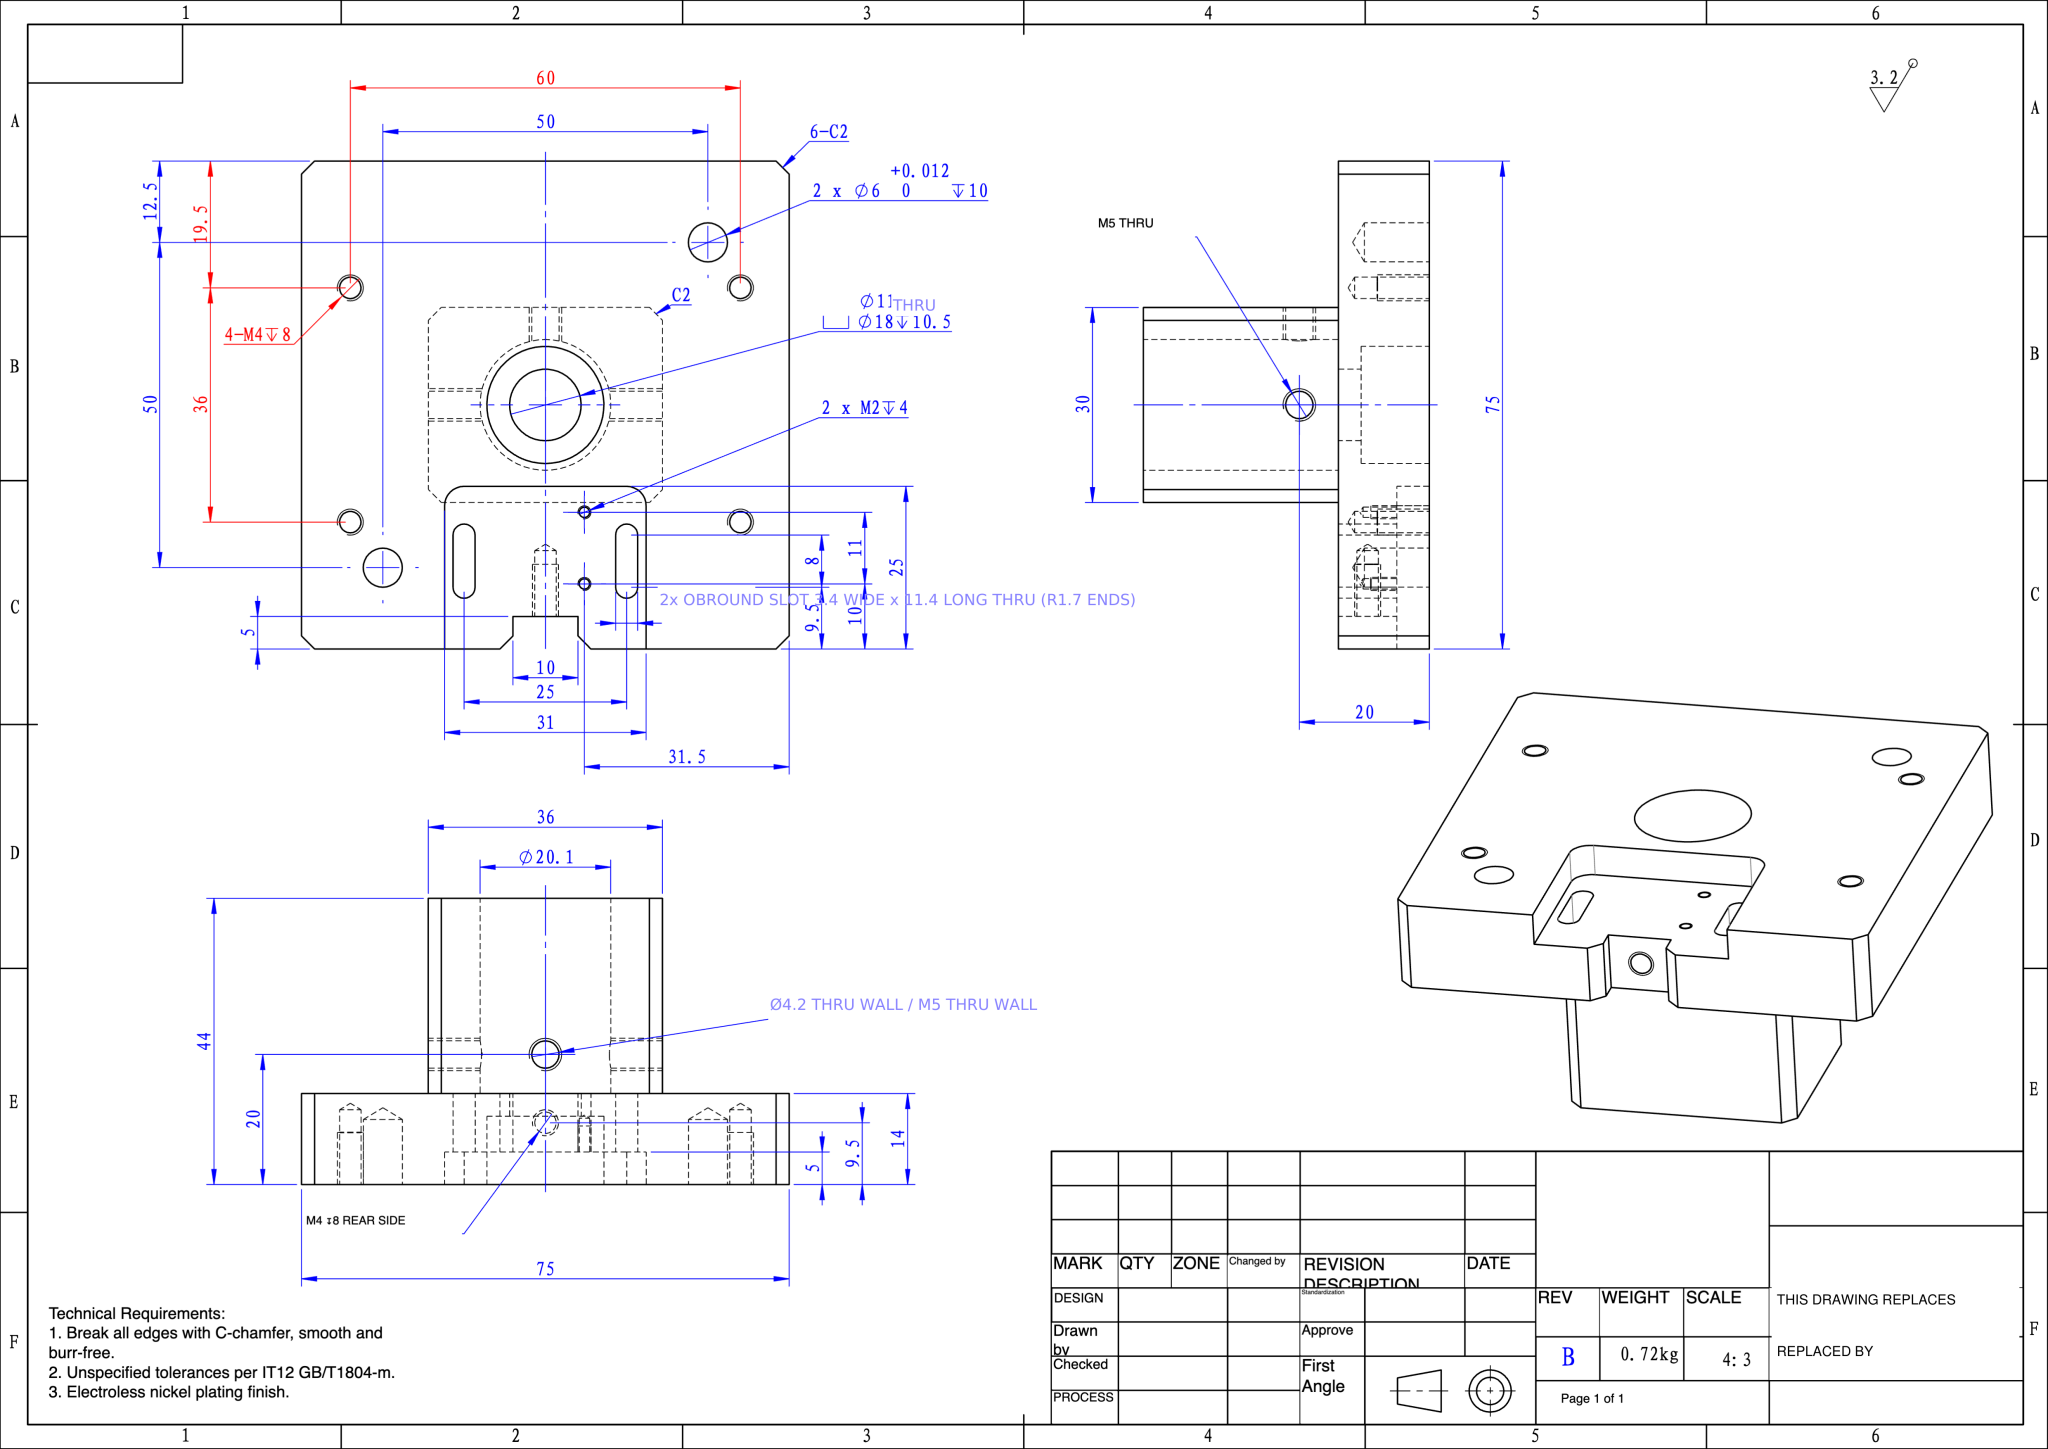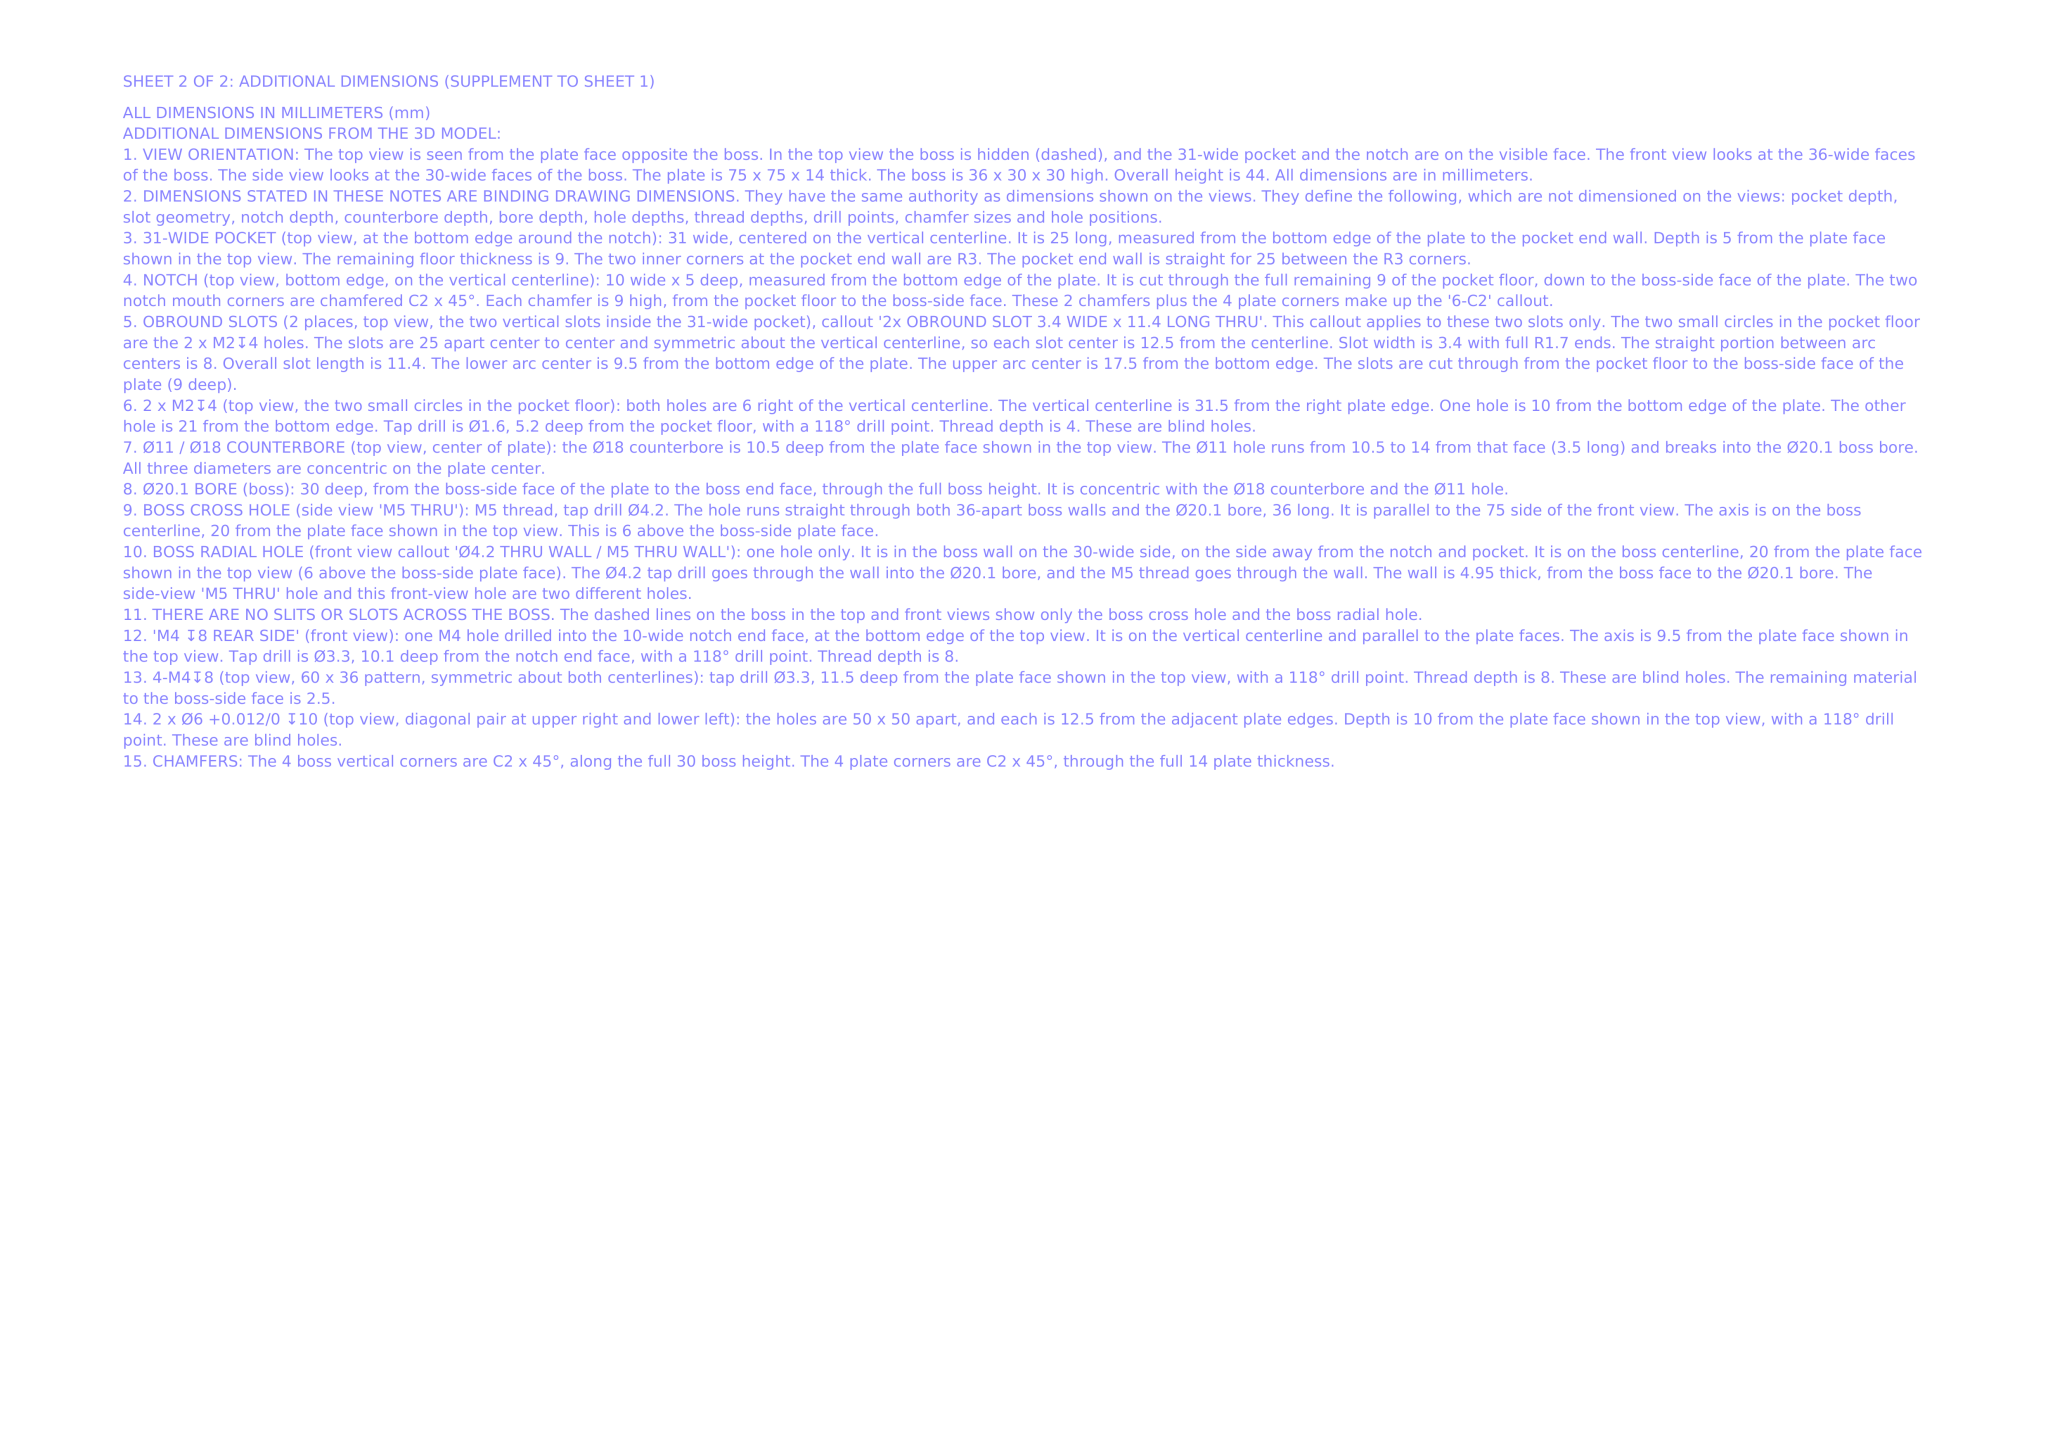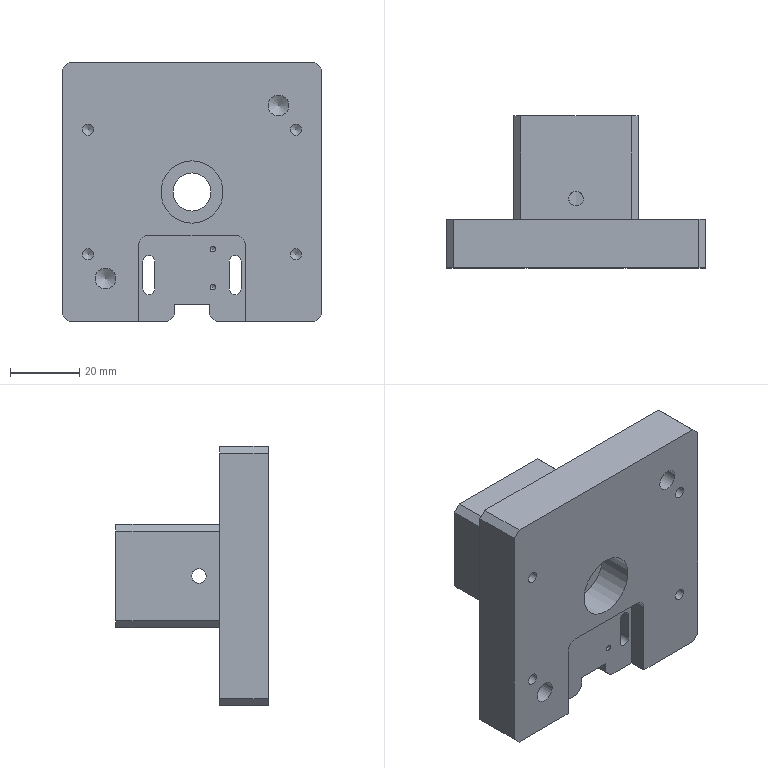Part | NX | mm | 1 solid | 65 faces | box 75 x 44 x 75 mm | volume 91873 mm3 | plane 35 | cylinder 21 | cone 9 | commonest cylinder face diameters 3.3 x5 6 x4 3.4 x4 4.2 x3 1.6 x2 20.1 x1 11 x1 18 x1